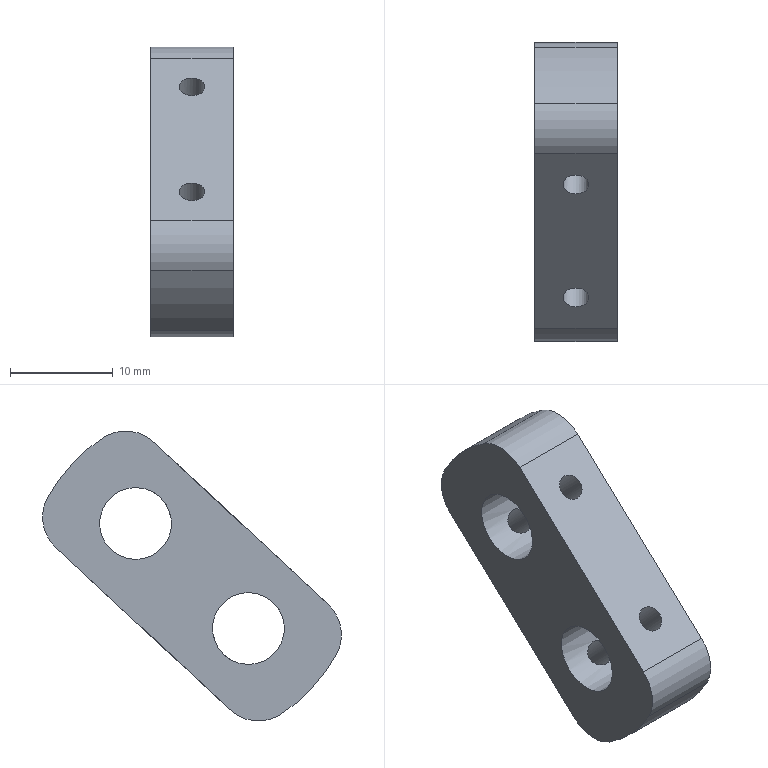Component | NX | 15A__27_2 | 1 solid | 16 faces | volume 2732 mm3 | cylinder 12 | plane 4 | commonest cylinder face diameters 8 x4 2.5 x4 32 x2 7 x2